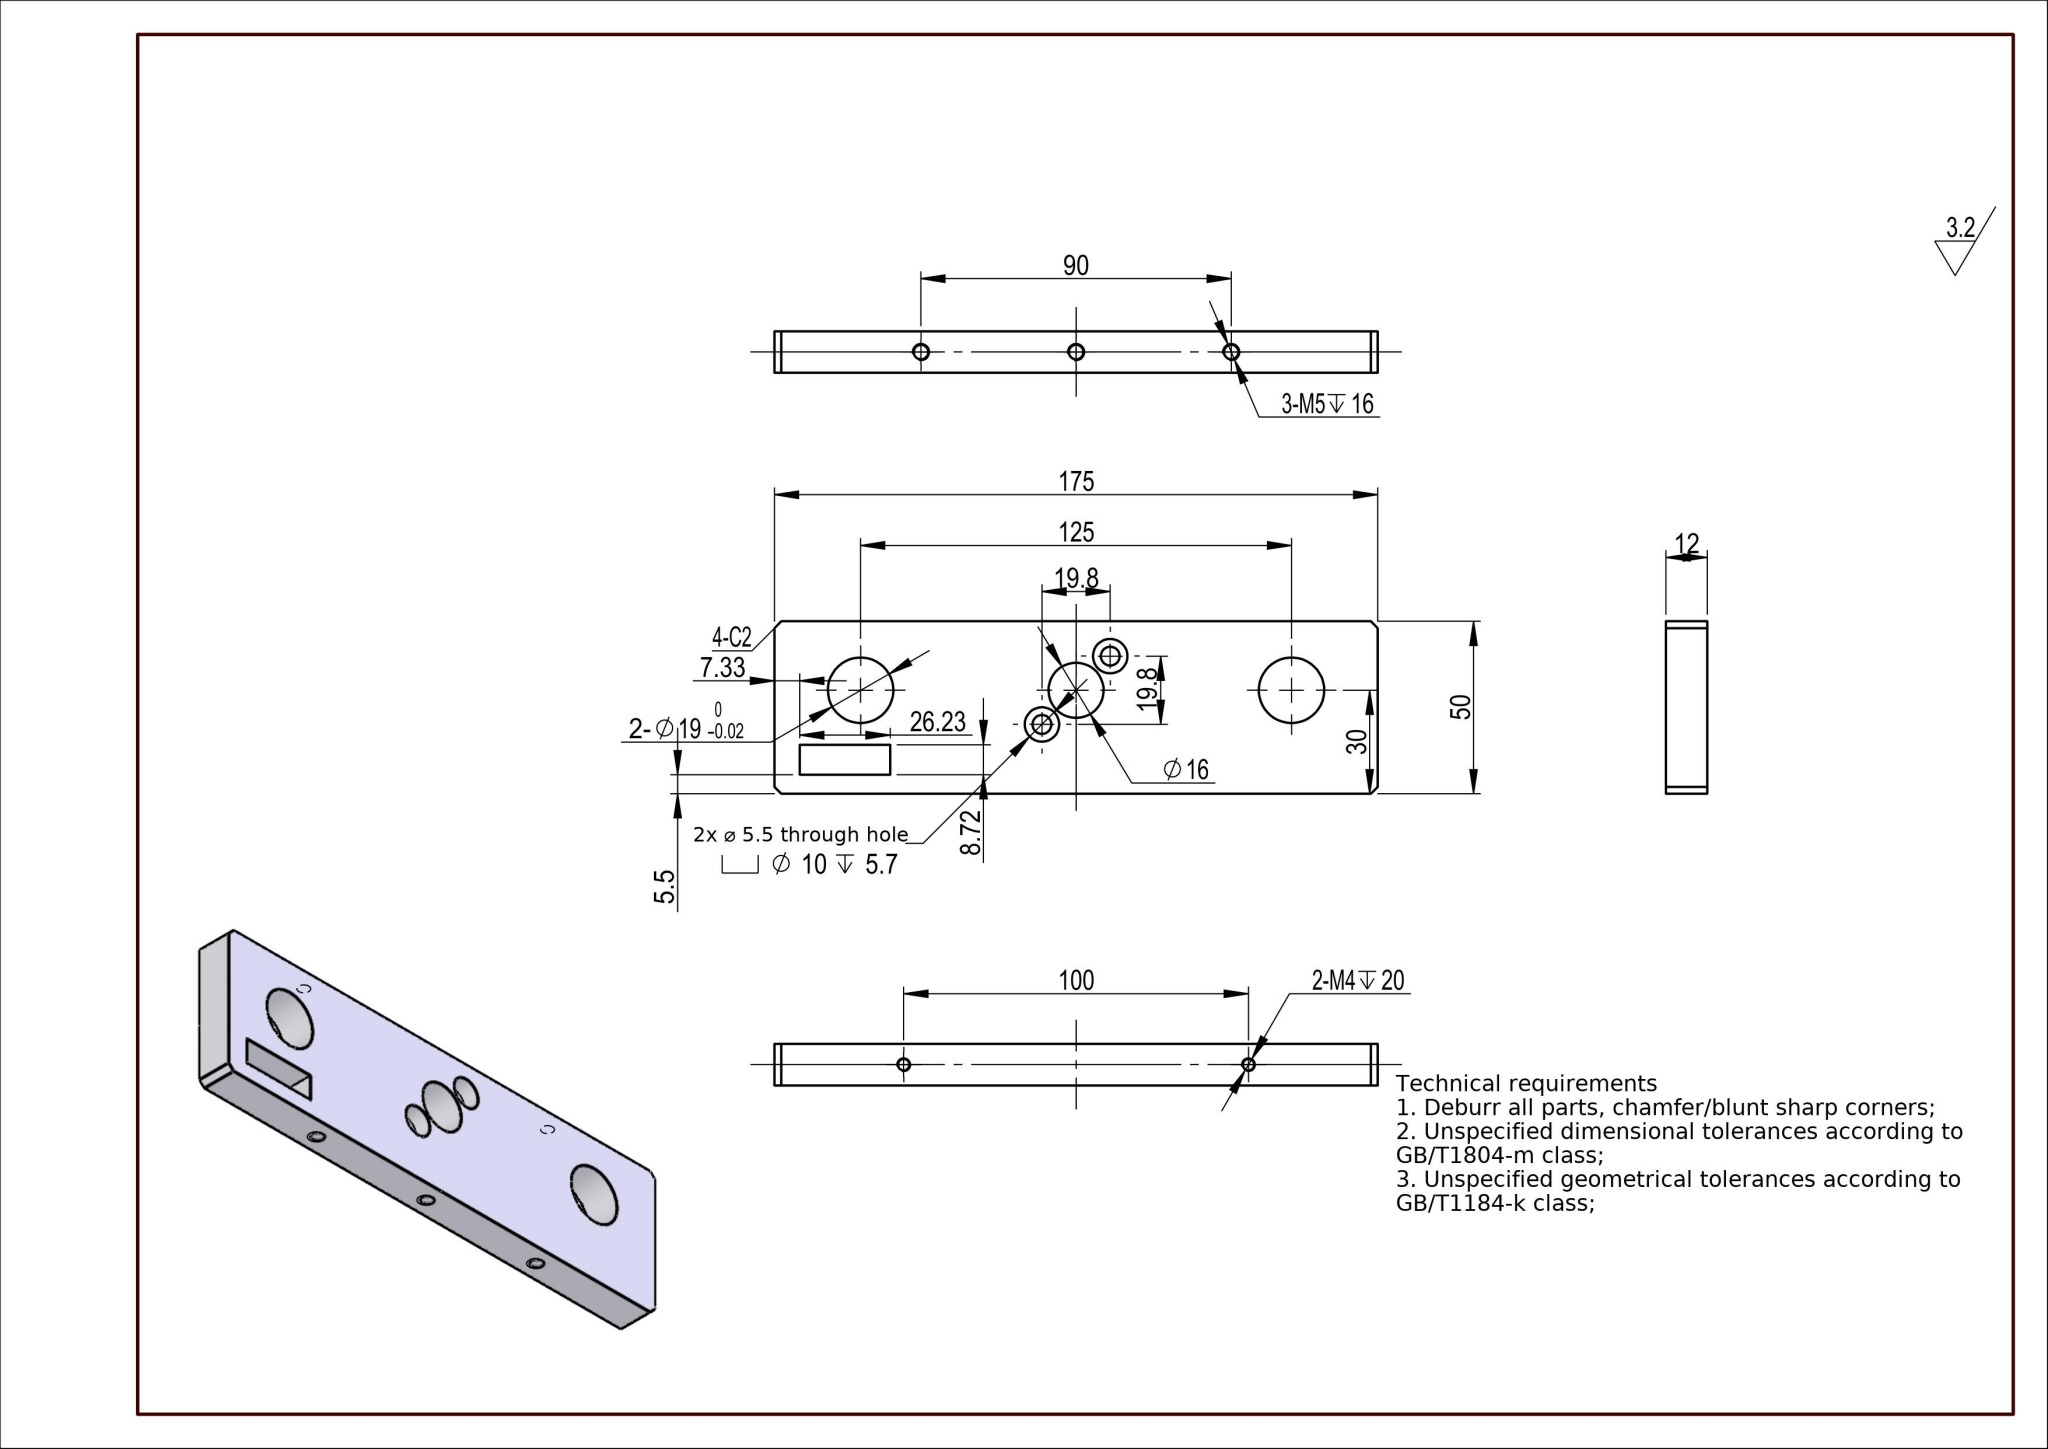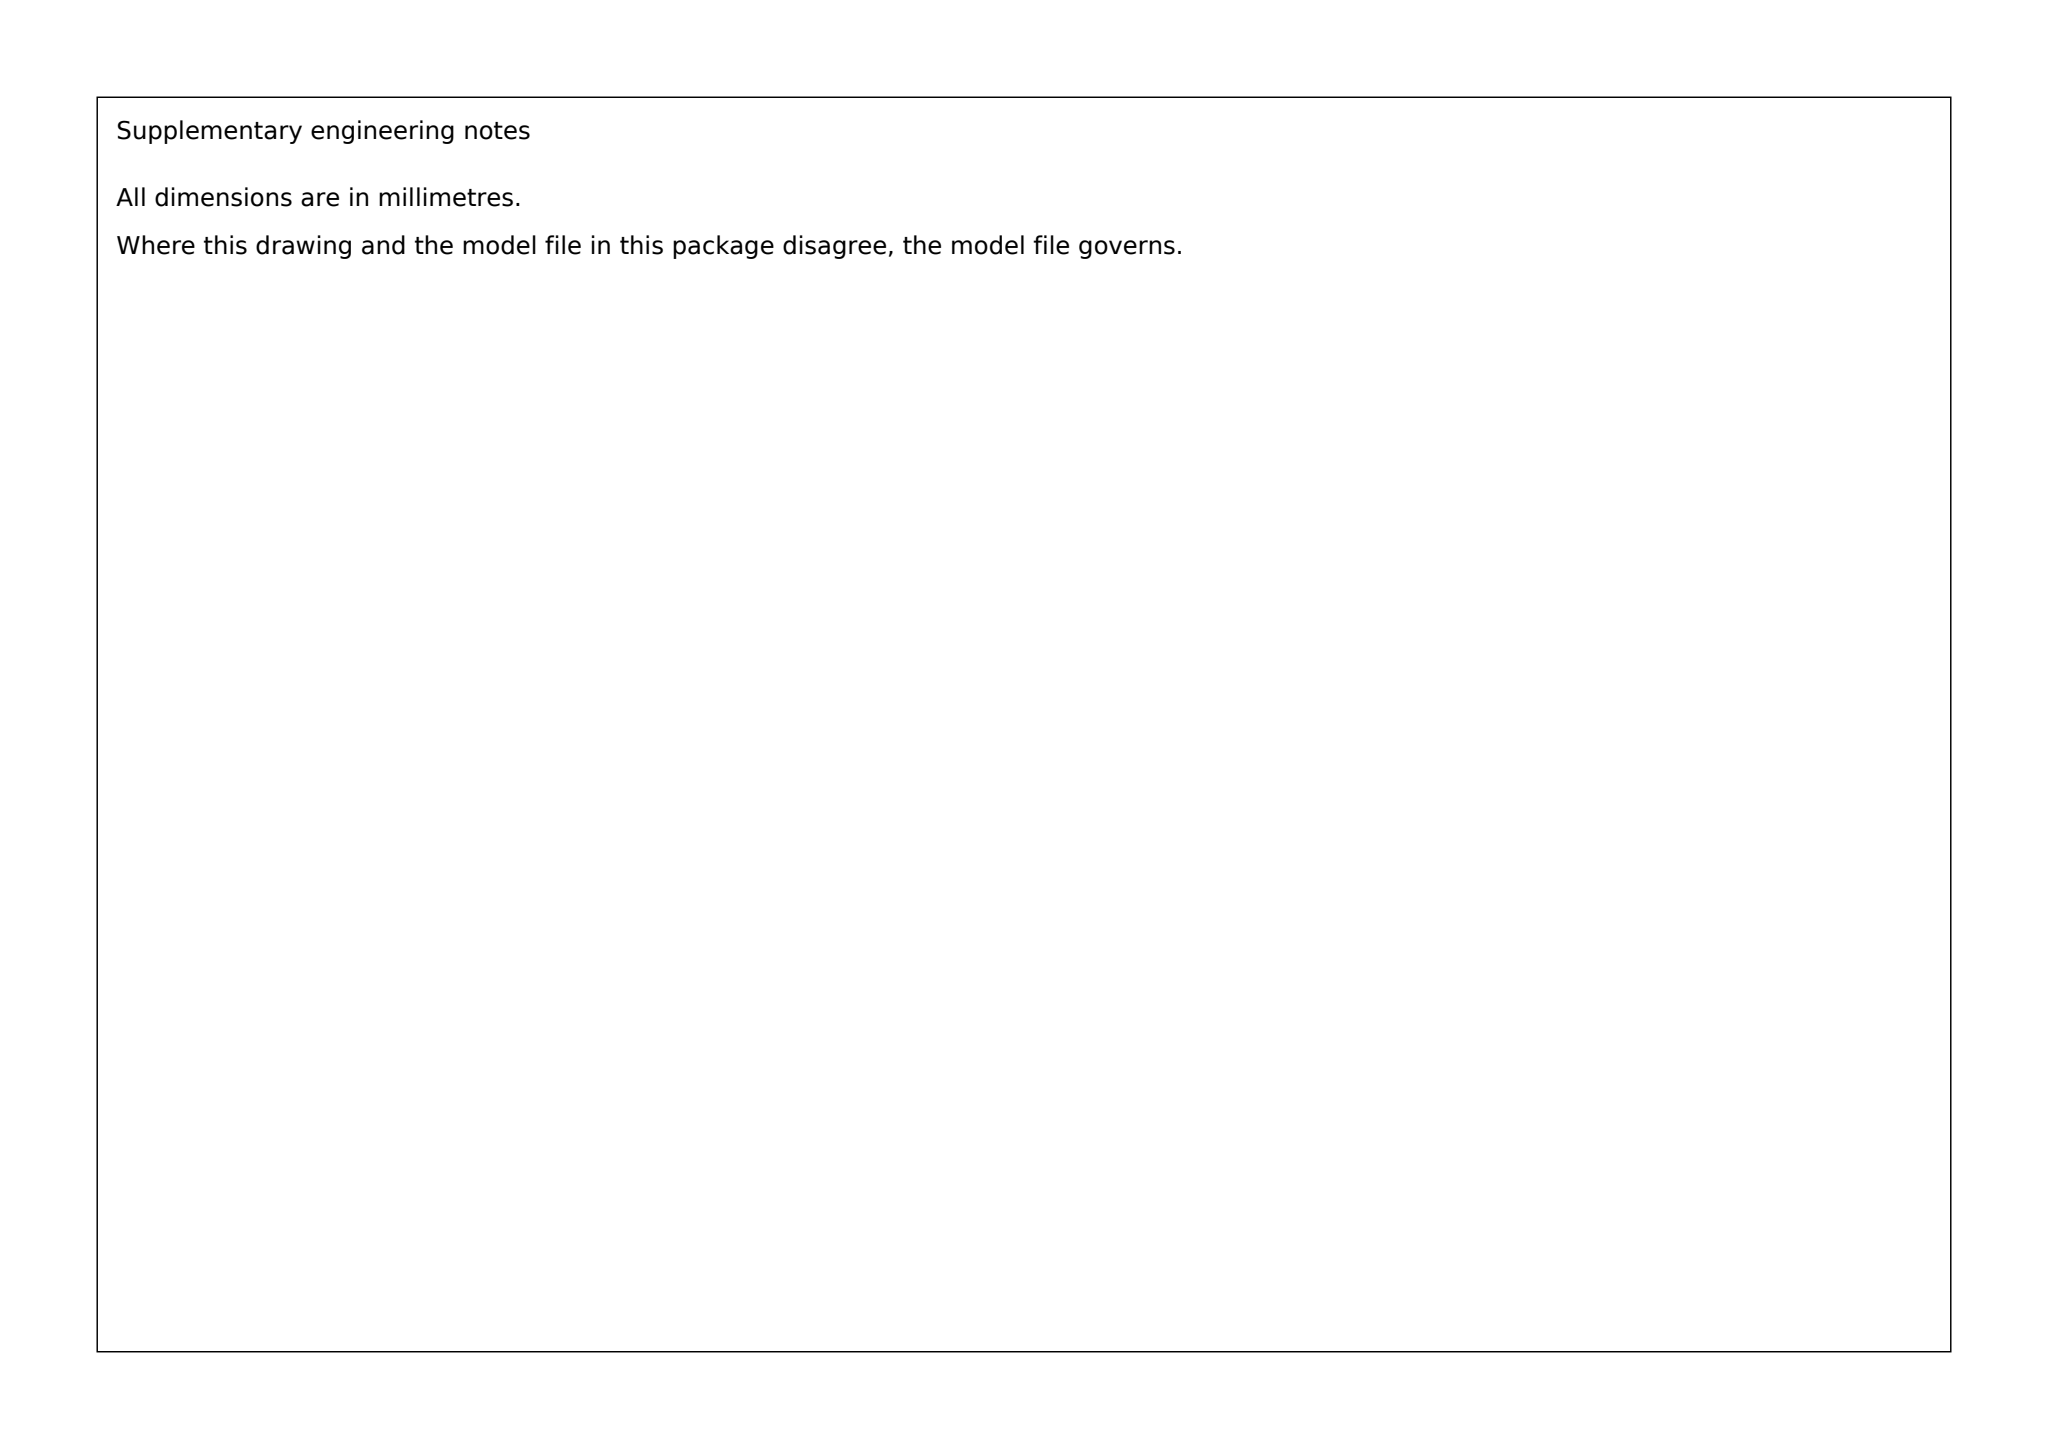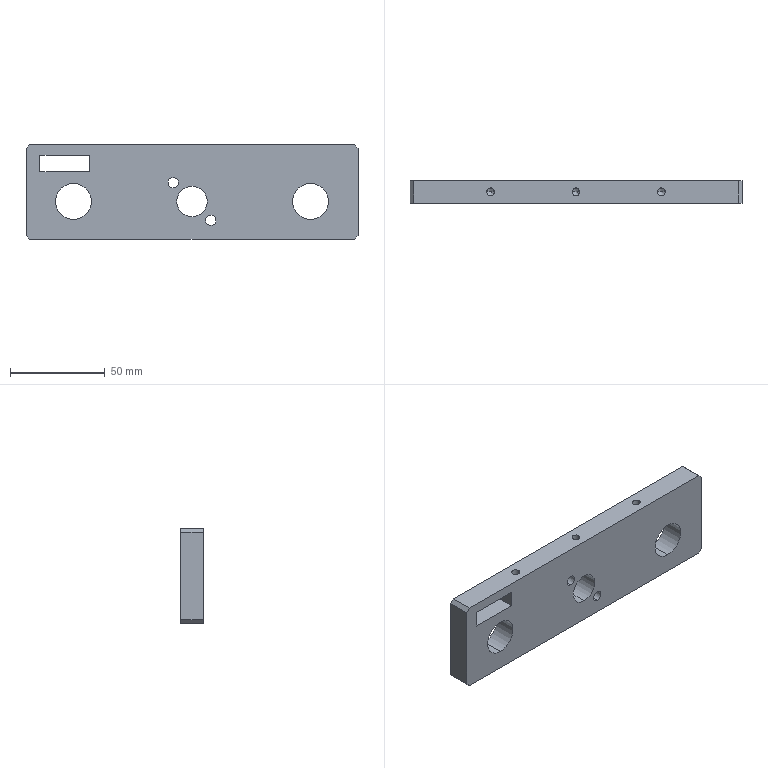Part | SolidWorks | mm | 1 solid | 50 faces | box 175 x 12 x 50 mm | volume 90752 mm3 | cylinder 24 | plane 16 | cone 10 | commonest cylinder face diameters 4.2 x6 3.3 x4 10 x4 5.5 x4 19 x4 16 x2
build123d program:
from build123d import *

# Parameters (mm, degrees)
SKETCH1_W                                            = 175
SKETCH1_H                                            = 50
BOSS_EXTRUDE1_DEPTH                                  = 6
M5_TAPPED_HOLE1_D                                    = 4.2
M5_TAPPED_HOLE1_DEPTH                                = 18.4
M5_TAPPED_HOLE1_TIP                                  = 1.262
SKETCH7_R                                            = 9.5
SKETCH7_R_2                                          = 8
CUT_EXTRUDE2_DEPTH                                   = 92.789
HOLE_SIZE_ACCORDING_TO_HEXAGON_SOCKET_HE_D           = 5.5
HOLE_SIZE_ACCORDING_TO_HEXAGON_SOCKET_HE_CBORE_D     = 10
HOLE_SIZE_ACCORDING_TO_HEXAGON_SOCKET_HE_CBORE_DEPTH = 5.7
M4_TAPPED_HOLE1_D                                    = 3.3
M4_TAPPED_HOLE1_DEPTH                                = 12.1
M4_TAPPED_HOLE1_TIP                                  = 0.9914
CHAMFER1_SIZE                                        = 2
SKETCH10_W                                           = 26.234
SKETCH10_H                                           = 8.718
CUT_EXTRUDE3_DEPTH                                   = 24


with BuildPart() as part:
    # Sketch1 → Boss-Extrude1 (new, symmetric)
    with BuildSketch(Plane(origin=(0, 0, 0), x_dir=(1, 0, 0), z_dir=(0, 1, 0))):
        Rectangle(SKETCH1_W, SKETCH1_H)
    extrude(amount=BOSS_EXTRUDE1_DEPTH, both=True)

    # M5 Tapped Hole1
    with Locations(Plane.XY.offset(25)):
        with Locations((-45, 0), (0, 0), (45, 0)):
            Hole(M5_TAPPED_HOLE1_D / 2, depth=M5_TAPPED_HOLE1_DEPTH)
            with Locations((0, 0, -(M5_TAPPED_HOLE1_DEPTH + M5_TAPPED_HOLE1_TIP / 2))):  # 118° drill point
                Cone(0, M5_TAPPED_HOLE1_D / 2, M5_TAPPED_HOLE1_TIP, mode=Mode.SUBTRACT)

    # Sketch7 → Cut-Extrude2 (cut, through all)
    with BuildSketch(Plane(origin=(0, 6, 0), x_dir=(1, 0, 0), z_dir=(0, 1, 0))):
        with Locations(Location((62.5, 5, 0), (0, 0, 270))):
            Circle(SKETCH7_R)
        with Locations(Location((-62.5, 5, 0), (0, 0, 270))):
            Circle(SKETCH7_R)
        with Locations(Location((0, 5, 0), (0, 0, 270))):
            Circle(SKETCH7_R_2)
    extrude(amount=-CUT_EXTRUDE2_DEPTH, mode=Mode.SUBTRACT)

    # Hole Size according to Hexagon Socket He (through all)
    with Locations(Plane(origin=(0, 6, 0), x_dir=(-1, 0, 0), z_dir=(0, 1, 0))):
        with Locations((9.899, 4.899), (-9.899, -14.899)):
            CounterBoreHole(HOLE_SIZE_ACCORDING_TO_HEXAGON_SOCKET_HE_D / 2, HOLE_SIZE_ACCORDING_TO_HEXAGON_SOCKET_HE_CBORE_D / 2, HOLE_SIZE_ACCORDING_TO_HEXAGON_SOCKET_HE_CBORE_DEPTH)

    # M4 Tapped Hole1
    with Locations(Plane(origin=(0, 0, -25), x_dir=(-1, 0, 0), z_dir=(0, 0, -1))):
        with Locations((-50, 0), (50, 0)):
            Hole(M4_TAPPED_HOLE1_D / 2, depth=M4_TAPPED_HOLE1_DEPTH)
            with Locations((0, 0, -(M4_TAPPED_HOLE1_DEPTH + M4_TAPPED_HOLE1_TIP / 2))):  # 118° drill point
                Cone(0, M4_TAPPED_HOLE1_D / 2, M4_TAPPED_HOLE1_TIP, mode=Mode.SUBTRACT)

    # Chamfer1
    chamfer1_edges = [part.edges().sort_by_distance(p)[0] for p in [
        (87.5, 0, 25),
        (-87.5, 0, 25),
        (-87.5, 0, -25),
        (87.5, 0, -25),
    ]]
    chamfer(chamfer1_edges, length=CHAMFER1_SIZE)

    # Sketch10 → Cut-Extrude3 (cut)
    with BuildSketch(Plane(origin=(0, 6, 0), x_dir=(1, 0, 0), z_dir=(0, 1, 0))):
        with Locations((-67.05, -15.139)):
            Rectangle(SKETCH10_W, SKETCH10_H)
    extrude(amount=-CUT_EXTRUDE3_DEPTH, mode=Mode.SUBTRACT)


solid = part.part